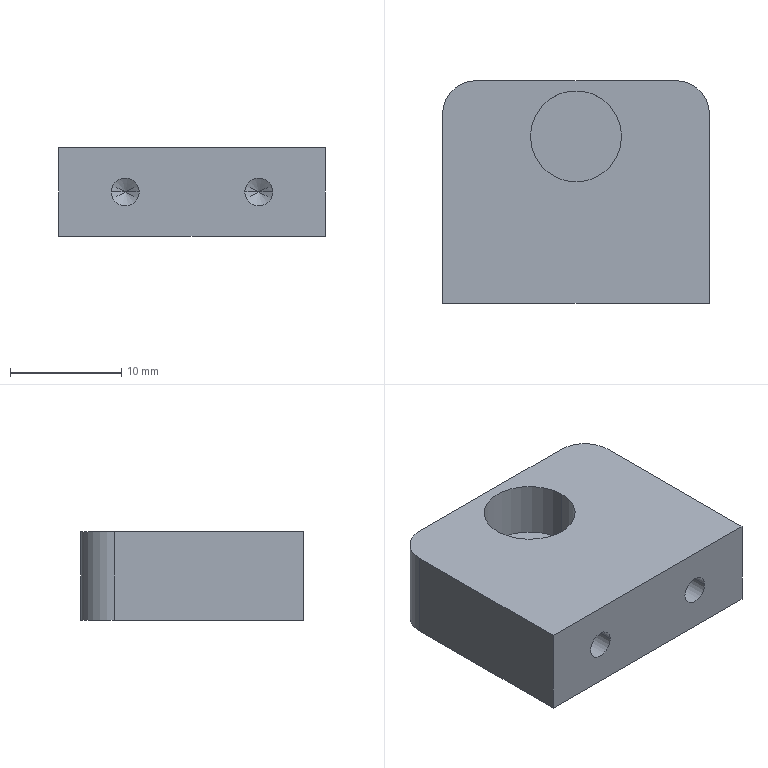Component | SolidWorks | SAWH02-03105A0MountingPlate5-7 | 1 solid | 19 faces | box 24 x 20 x 8 mm | volume 3469 mm3 | cylinder 8 | plane 7 | cone 4 | commonest cylinder face diameters 2.5 x4 8.2 x2 6 x2 | material 6061
build123d program:
from build123d import *

# Parameters (mm, degrees)
SKETCH1_W             = 20
SKETCH1_H             = 24
BOSS_EXTRUDE3_DEPTH   = 8
M3_TAPPED_HOLE1_D     = 2.5
M3_TAPPED_HOLE1_DEPTH = 7.5
M3_TAPPED_HOLE1_TIP   = 0.7511
SKETCH4_R             = 4.1
CUT_EXTRUDE1_DEPTH    = 5
FILLET1_R             = 3


with BuildPart() as part:
    # Sketch1 → Boss-Extrude3 (new body)
    with BuildSketch(Plane(origin=(0, 0, 0), x_dir=(1, 0, 0), z_dir=(0, 1, 0))):
        Rectangle(SKETCH1_W, SKETCH1_H)
    extrude(amount=BOSS_EXTRUDE3_DEPTH)

    # M3 Tapped Hole1
    with Locations(Plane.ZY.offset(10)):
        with Locations((-6, 4), (6, 4)):
            Hole(M3_TAPPED_HOLE1_D / 2, depth=M3_TAPPED_HOLE1_DEPTH)
            with Locations((0, 0, -(M3_TAPPED_HOLE1_DEPTH + M3_TAPPED_HOLE1_TIP / 2))):  # 118° drill point
                Cone(0, M3_TAPPED_HOLE1_D / 2, M3_TAPPED_HOLE1_TIP, mode=Mode.SUBTRACT)

    # Sketch4 → Cut-Extrude1 (cut)
    with BuildSketch(Plane(origin=(0, 8, 0), x_dir=(-1, 0, 0), z_dir=(0, -1, 0))):
        with Locations(Location((-5, 0, 0), (0, 0, 90))):
            Circle(SKETCH4_R)
    extrude(amount=CUT_EXTRUDE1_DEPTH, mode=Mode.SUBTRACT)

    # Fillet1
    fillet1_edges = [part.edges().sort_by_distance(p)[0] for p in [
        (10, 4, 12),
        (10, 4, -12),
    ]]
    fillet(fillet1_edges, radius=FILLET1_R)


solid = part.part

# Placed as in the assembly
solid = solid.moved(Location((81.51, -10.388, -138.792), (90, 90, 0)))
STEP:
#1=COLOUR_RGB('',0.7922,0.8196,0.9333);
#2=FILL_AREA_STYLE_COLOUR('',#1);
#3=FILL_AREA_STYLE('',(#2));
#4=SURFACE_STYLE_FILL_AREA(#3);
#5=SURFACE_SIDE_STYLE('',(#4));
#6=SURFACE_STYLE_USAGE(.BOTH.,#5);
#7=PRESENTATION_STYLE_ASSIGNMENT((#6));
#8=CARTESIAN_POINT('',(3.37,-0.2121,-5.346));
#9=VERTEX_POINT('',#8);
#10=CARTESIAN_POINT('',(3.048,-0.2121,-5.346));
#11=VERTEX_POINT('',#10);
#12=CARTESIAN_POINT('',(3.209,-0.2121,-5.346));
#13=DIRECTION('',(0.,0.,-1.));
#14=DIRECTION('',(-1.,-0.,0.));
#15=AXIS2_PLACEMENT_3D('',#12,#13,#14);
#16=CIRCLE('',#15,0.1614);
#17=EDGE_CURVE('',#9,#11,#16,.T.);
#18=ORIENTED_EDGE('',*,*,#17,.T.);
#19=CARTESIAN_POINT('',(3.048,-0.2121,-5.149));
#20=VERTEX_POINT('',#19);
#21=CARTESIAN_POINT('',(3.048,-0.2121,-5.346));
#22=DIRECTION('',(0.,-0.,1.));
#23=VECTOR('',#22,39.37);
#24=LINE('',#21,#23);
#25=EDGE_CURVE('',#11,#20,#24,.T.);
#26=ORIENTED_EDGE('',*,*,#25,.T.);
#27=CARTESIAN_POINT('',(3.37,-0.2121,-5.149));
#28=VERTEX_POINT('',#27);
#29=CARTESIAN_POINT('',(3.209,-0.2121,-5.149));
#30=DIRECTION('',(0.,0.,-1.));
#31=DIRECTION('',(-1.,-0.,0.));
#32=AXIS2_PLACEMENT_3D('',#29,#30,#31);
#33=CIRCLE('',#32,0.1614);
#34=EDGE_CURVE('',#28,#20,#33,.T.);
#35=ORIENTED_EDGE('',*,*,#34,.F.);
#36=CARTESIAN_POINT('',(3.37,-0.2121,-5.346));
#37=DIRECTION('',(0.,-0.,1.));
#38=VECTOR('',#37,39.37);
#39=LINE('',#36,#38);
#40=EDGE_CURVE('',#9,#28,#39,.T.);
#41=ORIENTED_EDGE('',*,*,#40,.F.);
#42=EDGE_LOOP('',(#18,#26,#35,#41));
#43=FACE_OUTER_BOUND('',#42,.T.);
#44=CARTESIAN_POINT('',(3.209,-0.2121,-5.346));
#45=DIRECTION('',(0.,-0.,1.));
#46=DIRECTION('',(1.,0.,0.));
#47=AXIS2_PLACEMENT_3D('',#44,#45,#46);
#48=CYLINDRICAL_SURFACE('',#47,0.1614);
#49=ADVANCED_FACE('',(#43),#48,.F.);
#50=CARTESIAN_POINT('',(2.924,-0.5074,-5.307));
#51=VERTEX_POINT('',#50);
#52=CARTESIAN_POINT('',(3.022,-0.5074,-5.307));
#53=VERTEX_POINT('',#52);
#54=CARTESIAN_POINT('',(2.973,-0.5074,-5.307));
#55=DIRECTION('',(0.,-1.,0.));
#56=DIRECTION('',(1.,0.,0.));
#57=AXIS2_PLACEMENT_3D('',#54,#55,#56);
#58=CIRCLE('',#57,0.04921);
#59=EDGE_CURVE('',#51,#53,#58,.T.);
#60=ORIENTED_EDGE('',*,*,#59,.F.);
#61=CARTESIAN_POINT('',(2.924,-0.8027,-5.307));
#62=VERTEX_POINT('',#61);
#63=CARTESIAN_POINT('',(2.924,-0.8027,-5.307));
#64=DIRECTION('',(0.,-1.,0.));
#65=VECTOR('',#64,39.37);
#66=LINE('',#63,#65);
#67=EDGE_CURVE('',#51,#62,#66,.T.);
#68=ORIENTED_EDGE('',*,*,#67,.T.);
#69=CARTESIAN_POINT('',(3.022,-0.8027,-5.307));
#70=VERTEX_POINT('',#69);
#71=CARTESIAN_POINT('',(2.973,-0.8027,-5.307));
#72=DIRECTION('',(0.,-1.,0.));
#73=DIRECTION('',(1.,0.,0.));
#74=AXIS2_PLACEMENT_3D('',#71,#72,#73);
#75=CIRCLE('',#74,0.04921);
#76=EDGE_CURVE('',#62,#70,#75,.T.);
#77=ORIENTED_EDGE('',*,*,#76,.T.);
#78=CARTESIAN_POINT('',(3.022,-0.8027,-5.307));
#79=DIRECTION('',(0.,-1.,0.));
#80=VECTOR('',#79,39.37);
#81=LINE('',#78,#80);
#82=EDGE_CURVE('',#53,#70,#81,.T.);
#83=ORIENTED_EDGE('',*,*,#82,.F.);
#84=EDGE_LOOP('',(#60,#68,#77,#83));
#85=FACE_OUTER_BOUND('',#84,.T.);
#86=CARTESIAN_POINT('',(2.973,-0.8027,-5.307));
#87=DIRECTION('',(0.,-1.,0.));
#88=DIRECTION('',(1.,0.,0.));
#89=AXIS2_PLACEMENT_3D('',#86,#87,#88);
#90=CYLINDRICAL_SURFACE('',#89,0.04921);
#91=ADVANCED_FACE('',(#85),#90,.F.);
#92=CARTESIAN_POINT('',(2.973,-0.4778,-5.307));
#93=VERTEX_POINT('',#92);
#94=CARTESIAN_POINT('',(3.022,-0.5074,-5.307));
#95=DIRECTION('',(0.8572,-0.515,0.));
#96=VECTOR('',#95,39.37);
#97=LINE('',#94,#96);
#98=EDGE_CURVE('',#93,#53,#97,.T.);
#99=ORIENTED_EDGE('',*,*,#98,.F.);
#100=CARTESIAN_POINT('',(2.924,-0.5074,-5.307));
#101=DIRECTION('',(-0.8572,-0.515,0.));
#102=VECTOR('',#101,39.37);
#103=LINE('',#100,#102);
#104=EDGE_CURVE('',#93,#51,#103,.T.);
#105=ORIENTED_EDGE('',*,*,#104,.T.);
#106=ORIENTED_EDGE('',*,*,#59,.T.);
#107=EDGE_LOOP('',(#99,#105,#106));
#108=FACE_OUTER_BOUND('',#107,.T.);
#109=CARTESIAN_POINT('',(2.973,-0.5074,-5.307));
#110=DIRECTION('',(0.,-1.,0.));
#111=DIRECTION('',(1.,0.,0.));
#112=AXIS2_PLACEMENT_3D('',#109,#110,#111);
#113=CONICAL_SURFACE('',#112,0.04921,1.03);
#114=ADVANCED_FACE('',(#108),#113,.F.);
#115=CARTESIAN_POINT('',(3.396,-0.5074,-5.307));
#116=VERTEX_POINT('',#115);
#117=CARTESIAN_POINT('',(3.494,-0.5074,-5.307));
#118=VERTEX_POINT('',#117);
#119=CARTESIAN_POINT('',(3.445,-0.5074,-5.307));
#120=DIRECTION('',(0.,-1.,0.));
#121=DIRECTION('',(1.,0.,0.));
#122=AXIS2_PLACEMENT_3D('',#119,#120,#121);
#123=CIRCLE('',#122,0.04921);
#124=EDGE_CURVE('',#116,#118,#123,.T.);
#125=ORIENTED_EDGE('',*,*,#124,.F.);
#126=CARTESIAN_POINT('',(3.396,-0.8027,-5.307));
#127=VERTEX_POINT('',#126);
#128=CARTESIAN_POINT('',(3.396,-0.8027,-5.307));
#129=DIRECTION('',(0.,-1.,0.));
#130=VECTOR('',#129,39.37);
#131=LINE('',#128,#130);
#132=EDGE_CURVE('',#116,#127,#131,.T.);
#133=ORIENTED_EDGE('',*,*,#132,.T.);
#134=CARTESIAN_POINT('',(3.494,-0.8027,-5.307));
#135=VERTEX_POINT('',#134);
#136=CARTESIAN_POINT('',(3.445,-0.8027,-5.307));
#137=DIRECTION('',(0.,-1.,0.));
#138=DIRECTION('',(1.,0.,0.));
#139=AXIS2_PLACEMENT_3D('',#136,#137,#138);
#140=CIRCLE('',#139,0.04921);
#141=EDGE_CURVE('',#127,#135,#140,.T.);
#142=ORIENTED_EDGE('',*,*,#141,.T.);
#143=CARTESIAN_POINT('',(3.494,-0.8027,-5.307));
#144=DIRECTION('',(0.,-1.,0.));
#145=VECTOR('',#144,39.37);
#146=LINE('',#143,#145);
#147=EDGE_CURVE('',#118,#135,#146,.T.);
#148=ORIENTED_EDGE('',*,*,#147,.F.);
#149=EDGE_LOOP('',(#125,#133,#142,#148));
#150=FACE_OUTER_BOUND('',#149,.T.);
#151=CARTESIAN_POINT('',(3.445,-0.8027,-5.307));
#152=DIRECTION('',(0.,-1.,0.));
#153=DIRECTION('',(1.,0.,0.));
#154=AXIS2_PLACEMENT_3D('',#151,#152,#153);
#155=CYLINDRICAL_SURFACE('',#154,0.04921);
#156=ADVANCED_FACE('',(#150),#155,.F.);
#157=CARTESIAN_POINT('',(3.445,-0.4778,-5.307));
#158=VERTEX_POINT('',#157);
#159=CARTESIAN_POINT('',(3.494,-0.5074,-5.307));
#160=DIRECTION('',(0.8572,-0.515,0.));
#161=VECTOR('',#160,39.37);
#162=LINE('',#159,#161);
#163=EDGE_CURVE('',#158,#118,#162,.T.);
#164=ORIENTED_EDGE('',*,*,#163,.F.);
#165=CARTESIAN_POINT('',(3.396,-0.5074,-5.307));
#166=DIRECTION('',(-0.8572,-0.515,0.));
#167=VECTOR('',#166,39.37);
#168=LINE('',#165,#167);
#169=EDGE_CURVE('',#158,#116,#168,.T.);
#170=ORIENTED_EDGE('',*,*,#169,.T.);
#171=ORIENTED_EDGE('',*,*,#124,.T.);
#172=EDGE_LOOP('',(#164,#170,#171));
#173=FACE_OUTER_BOUND('',#172,.T.);
#174=CARTESIAN_POINT('',(3.445,-0.5074,-5.307));
#175=DIRECTION('',(0.,-1.,0.));
#176=DIRECTION('',(1.,0.,0.));
#177=AXIS2_PLACEMENT_3D('',#174,#175,#176);
#178=CONICAL_SURFACE('',#177,0.04921,1.03);
#179=ADVANCED_FACE('',(#173),#178,.F.);
#180=CARTESIAN_POINT('',(3.563,-0.01526,-5.149));
#181=VERTEX_POINT('',#180);
#182=CARTESIAN_POINT('',(2.855,-0.01526,-5.149));
#183=VERTEX_POINT('',#182);
#184=CARTESIAN_POINT('',(3.682,-0.01526,-5.149));
#185=DIRECTION('',(-1.,-0.,0.));
#186=VECTOR('',#185,39.37);
#187=LINE('',#184,#186);
#188=EDGE_CURVE('',#181,#183,#187,.T.);
#189=ORIENTED_EDGE('',*,*,#188,.F.);
#190=CARTESIAN_POINT('',(3.563,-0.01526,-5.464));
#191=VERTEX_POINT('',#190);
#192=CARTESIAN_POINT('',(3.563,-0.01526,-5.149));
#193=DIRECTION('',(0.,0.,-1.));
#194=VECTOR('',#193,39.37);
#195=LINE('',#192,#194);
#196=EDGE_CURVE('',#181,#191,#195,.T.);
#197=ORIENTED_EDGE('',*,*,#196,.T.);
#198=CARTESIAN_POINT('',(2.855,-0.01526,-5.464));
#199=VERTEX_POINT('',#198);
#200=CARTESIAN_POINT('',(3.682,-0.01526,-5.464));
#201=DIRECTION('',(-1.,-0.,0.));
#202=VECTOR('',#201,39.37);
#203=LINE('',#200,#202);
#204=EDGE_CURVE('',#191,#199,#203,.T.);
#205=ORIENTED_EDGE('',*,*,#204,.T.);
#206=CARTESIAN_POINT('',(2.855,-0.01526,-5.149));
#207=DIRECTION('',(0.,-0.,1.));
#208=VECTOR('',#207,39.37);
#209=LINE('',#206,#208);
#210=EDGE_CURVE('',#199,#183,#209,.T.);
#211=ORIENTED_EDGE('',*,*,#210,.T.);
#212=EDGE_LOOP('',(#189,#197,#205,#211));
#213=FACE_OUTER_BOUND('',#212,.T.);
#214=CARTESIAN_POINT('',(3.682,-0.01526,-5.149));
#215=DIRECTION('',(0.,-1.,0.));
#216=DIRECTION('',(1.,0.,0.));
#217=AXIS2_PLACEMENT_3D('',#214,#215,#216);
#218=PLANE('',#217);
#219=ADVANCED_FACE('',(#213),#218,.F.);
#220=CARTESIAN_POINT('',(2.737,-0.1334,-5.149));
#221=VERTEX_POINT('',#220);
#222=CARTESIAN_POINT('',(2.737,-0.8027,-5.149));
#223=VERTEX_POINT('',#222);
#224=CARTESIAN_POINT('',(2.737,-0.8027,-5.149));
#225=DIRECTION('',(0.,-1.,0.));
#226=VECTOR('',#225,39.37);
#227=LINE('',#224,#226);
#228=EDGE_CURVE('',#221,#223,#227,.T.);
#229=ORIENTED_EDGE('',*,*,#228,.F.);
#230=CARTESIAN_POINT('',(2.737,-0.1334,-5.464));
#231=VERTEX_POINT('',#230);
#232=CARTESIAN_POINT('',(2.737,-0.1334,-5.149));
#233=DIRECTION('',(0.,0.,-1.));
#234=VECTOR('',#233,39.37);
#235=LINE('',#232,#234);
#236=EDGE_CURVE('',#221,#231,#235,.T.);
#237=ORIENTED_EDGE('',*,*,#236,.T.);
#238=CARTESIAN_POINT('',(2.737,-0.8027,-5.464));
#239=VERTEX_POINT('',#238);
#240=CARTESIAN_POINT('',(2.737,-0.8027,-5.464));
#241=DIRECTION('',(0.,-1.,0.));
#242=VECTOR('',#241,39.37);
#243=LINE('',#240,#242);
#244=EDGE_CURVE('',#231,#239,#243,.T.);
#245=ORIENTED_EDGE('',*,*,#244,.T.);
#246=CARTESIAN_POINT('',(2.737,-0.8027,-5.149));
#247=DIRECTION('',(0.,0.,-1.));
#248=VECTOR('',#247,39.37);
#249=LINE('',#246,#248);
#250=EDGE_CURVE('',#223,#239,#249,.T.);
#251=ORIENTED_EDGE('',*,*,#250,.F.);
#252=EDGE_LOOP('',(#229,#237,#245,#251));
#253=FACE_OUTER_BOUND('',#252,.T.);
#254=CARTESIAN_POINT('',(2.737,-0.8027,-5.149));
#255=DIRECTION('',(1.,0.,0.));
#256=DIRECTION('',(-0.,1.,-0.));
#257=AXIS2_PLACEMENT_3D('',#254,#255,#256);
#258=PLANE('',#257);
#259=ADVANCED_FACE('',(#253),#258,.F.);
#260=CARTESIAN_POINT('',(2.973,-0.8027,-5.307));
#261=DIRECTION('',(0.,-1.,0.));
#262=DIRECTION('',(1.,0.,0.));
#263=AXIS2_PLACEMENT_3D('',#260,#261,#262);
#264=CIRCLE('',#263,0.04921);
#265=EDGE_CURVE('',#70,#62,#264,.T.);
#266=ORIENTED_EDGE('',*,*,#265,.F.);
#267=ORIENTED_EDGE('',*,*,#76,.F.);
#268=EDGE_LOOP('',(#266,#267));
#269=FACE_BOUND('',#268,.T.);
#270=CARTESIAN_POINT('',(3.445,-0.8027,-5.307));
#271=DIRECTION('',(0.,-1.,0.));
#272=DIRECTION('',(1.,0.,0.));
#273=AXIS2_PLACEMENT_3D('',#270,#271,#272);
#274=CIRCLE('',#273,0.04921);
#275=EDGE_CURVE('',#135,#127,#274,.T.);
#276=ORIENTED_EDGE('',*,*,#275,.F.);
#277=ORIENTED_EDGE('',*,*,#141,.F.);
#278=EDGE_LOOP('',(#276,#277));
#279=FACE_BOUND('',#278,.T.);
#280=CARTESIAN_POINT('',(3.682,-0.8027,-5.464));
#281=VERTEX_POINT('',#280);
#282=CARTESIAN_POINT('',(3.682,-0.8027,-5.464));
#283=DIRECTION('',(1.,0.,0.));
#284=VECTOR('',#283,39.37);
#285=LINE('',#282,#284);
#286=EDGE_CURVE('',#239,#281,#285,.T.);
#287=ORIENTED_EDGE('',*,*,#286,.T.);
#288=CARTESIAN_POINT('',(3.682,-0.8027,-5.149));
#289=VERTEX_POINT('',#288);
#290=CARTESIAN_POINT('',(3.682,-0.8027,-5.149));
#291=DIRECTION('',(0.,0.,-1.));
#292=VECTOR('',#291,39.37);
#293=LINE('',#290,#292);
#294=EDGE_CURVE('',#289,#281,#293,.T.);
#295=ORIENTED_EDGE('',*,*,#294,.F.);
#296=CARTESIAN_POINT('',(3.682,-0.8027,-5.149));
#297=DIRECTION('',(1.,0.,0.));
#298=VECTOR('',#297,39.37);
#299=LINE('',#296,#298);
#300=EDGE_CURVE('',#223,#289,#299,.T.);
#301=ORIENTED_EDGE('',*,*,#300,.F.);
#302=ORIENTED_EDGE('',*,*,#250,.T.);
#303=EDGE_LOOP('',(#287,#295,#301,#302));
#304=FACE_OUTER_BOUND('',#303,.T.);
#305=CARTESIAN_POINT('',(3.682,-0.8027,-5.149));
#306=DIRECTION('',(-0.,1.,-0.));
#307=DIRECTION('',(-1.,-0.,0.));
#308=AXIS2_PLACEMENT_3D('',#305,#306,#307);
#309=PLANE('',#308);
#310=ADVANCED_FACE('',(#269,#279,#304),#309,.F.);
#311=CARTESIAN_POINT('',(3.682,-0.1334,-5.464));
#312=VERTEX_POINT('',#311);
#313=CARTESIAN_POINT('',(3.682,-0.8027,-5.464));
#314=DIRECTION('',(-0.,1.,-0.));
#315=VECTOR('',#314,39.37);
#316=LINE('',#313,#315);
#317=EDGE_CURVE('',#281,#312,#316,.T.);
#318=ORIENTED_EDGE('',*,*,#317,.T.);
#319=CARTESIAN_POINT('',(3.682,-0.1334,-5.149));
#320=VERTEX_POINT('',#319);
#321=CARTESIAN_POINT('',(3.682,-0.1334,-5.149));
#322=DIRECTION('',(0.,-0.,1.));
#323=VECTOR('',#322,39.37);
#324=LINE('',#321,#323);
#325=EDGE_CURVE('',#312,#320,#324,.T.);
#326=ORIENTED_EDGE('',*,*,#325,.T.);
#327=CARTESIAN_POINT('',(3.682,-0.8027,-5.149));
#328=DIRECTION('',(-0.,1.,-0.));
#329=VECTOR('',#328,39.37);
#330=LINE('',#327,#329);
#331=EDGE_CURVE('',#289,#320,#330,.T.);
#332=ORIENTED_EDGE('',*,*,#331,.F.);
#333=ORIENTED_EDGE('',*,*,#294,.T.);
#334=EDGE_LOOP('',(#318,#326,#332,#333));
#335=FACE_OUTER_BOUND('',#334,.T.);
#336=CARTESIAN_POINT('',(3.682,-0.8027,-5.149));
#337=DIRECTION('',(-1.,-0.,-0.));
#338=DIRECTION('',(0.,-1.,0.));
#339=AXIS2_PLACEMENT_3D('',#336,#337,#338);
#340=PLANE('',#339);
#341=ADVANCED_FACE('',(#335),#340,.F.);
#342=ORIENTED_EDGE('',*,*,#34,.T.);
#343=CARTESIAN_POINT('',(3.209,-0.2121,-5.149));
#344=DIRECTION('',(0.,0.,-1.));
#345=DIRECTION('',(-1.,-0.,0.));
#346=AXIS2_PLACEMENT_3D('',#343,#344,#345);
#347=CIRCLE('',#346,0.1614);
#348=EDGE_CURVE('',#20,#28,#347,.T.);
#349=ORIENTED_EDGE('',*,*,#348,.T.);
#350=EDGE_LOOP('',(#342,#349));
#351=FACE_BOUND('',#350,.T.);
#352=ORIENTED_EDGE('',*,*,#331,.T.);
#353=CARTESIAN_POINT('',(3.563,-0.1334,-5.149));
#354=DIRECTION('',(0.,-0.,1.));
#355=DIRECTION('',(-1.,-0.,0.));
#356=AXIS2_PLACEMENT_3D('',#353,#354,#355);
#357=CIRCLE('',#356,0.1181);
#358=EDGE_CURVE('',#320,#181,#357,.T.);
#359=ORIENTED_EDGE('',*,*,#358,.T.);
#360=ORIENTED_EDGE('',*,*,#188,.T.);
#361=CARTESIAN_POINT('',(2.855,-0.1334,-5.149));
#362=DIRECTION('',(0.,-0.,1.));
#363=DIRECTION('',(-1.,0.,0.));
#364=AXIS2_PLACEMENT_3D('',#361,#362,#363);
#365=CIRCLE('',#364,0.1181);
#366=EDGE_CURVE('',#183,#221,#365,.T.);
#367=ORIENTED_EDGE('',*,*,#366,.T.);
#368=ORIENTED_EDGE('',*,*,#228,.T.);
#369=ORIENTED_EDGE('',*,*,#300,.T.);
#370=EDGE_LOOP('',(#352,#359,#360,#367,#368,#369));
#371=FACE_OUTER_BOUND('',#370,.T.);
#372=CARTESIAN_POINT('',(3.209,-0.409,-5.149));
#373=DIRECTION('',(-0.,0.,-1.));
#374=DIRECTION('',(-1.,-0.,0.));
#375=AXIS2_PLACEMENT_3D('',#372,#373,#374);
#376=PLANE('',#375);
#377=ADVANCED_FACE('',(#351,#371),#376,.F.);
#378=ORIENTED_EDGE('',*,*,#204,.F.);
#379=CARTESIAN_POINT('',(3.563,-0.1334,-5.464));
#380=DIRECTION('',(0.,0.,-1.));
#381=DIRECTION('',(-1.,-0.,0.));
#382=AXIS2_PLACEMENT_3D('',#379,#380,#381);
#383=CIRCLE('',#382,0.1181);
#384=EDGE_CURVE('',#191,#312,#383,.T.);
#385=ORIENTED_EDGE('',*,*,#384,.T.);
#386=ORIENTED_EDGE('',*,*,#317,.F.);
#387=ORIENTED_EDGE('',*,*,#286,.F.);
#388=ORIENTED_EDGE('',*,*,#244,.F.);
#389=CARTESIAN_POINT('',(2.855,-0.1334,-5.464));
#390=DIRECTION('',(0.,0.,-1.));
#391=DIRECTION('',(-1.,-0.,0.));
#392=AXIS2_PLACEMENT_3D('',#389,#390,#391);
#393=CIRCLE('',#392,0.1181);
#394=EDGE_CURVE('',#231,#199,#393,.T.);
#395=ORIENTED_EDGE('',*,*,#394,.T.);
#396=EDGE_LOOP('',(#378,#385,#386,#387,#388,#395));
#397=FACE_OUTER_BOUND('',#396,.T.);
#398=CARTESIAN_POINT('',(3.209,-0.409,-5.464));
#399=DIRECTION('',(-0.,0.,-1.));
#400=DIRECTION('',(-1.,-0.,0.));
#401=AXIS2_PLACEMENT_3D('',#398,#399,#400);
#402=PLANE('',#401);
#403=ADVANCED_FACE('',(#397),#402,.T.);
#404=ORIENTED_EDGE('',*,*,#169,.F.);
#405=ORIENTED_EDGE('',*,*,#163,.T.);
#406=CARTESIAN_POINT('',(3.445,-0.5074,-5.307));
#407=DIRECTION('',(0.,-1.,0.));
#408=DIRECTION('',(1.,0.,0.));
#409=AXIS2_PLACEMENT_3D('',#406,#407,#408);
#410=CIRCLE('',#409,0.04921);
#411=EDGE_CURVE('',#118,#116,#410,.T.);
#412=ORIENTED_EDGE('',*,*,#411,.T.);
#413=EDGE_LOOP('',(#404,#405,#412));
#414=FACE_OUTER_BOUND('',#413,.T.);
#415=CARTESIAN_POINT('',(3.445,-0.5074,-5.307));
#416=DIRECTION('',(0.,-1.,0.));
#417=DIRECTION('',(1.,0.,0.));
#418=AXIS2_PLACEMENT_3D('',#415,#416,#417);
#419=CONICAL_SURFACE('',#418,0.04921,1.03);
#420=ADVANCED_FACE('',(#414),#419,.F.);
#421=ORIENTED_EDGE('',*,*,#132,.F.);
#422=ORIENTED_EDGE('',*,*,#411,.F.);
#423=ORIENTED_EDGE('',*,*,#147,.T.);
#424=ORIENTED_EDGE('',*,*,#275,.T.);
#425=EDGE_LOOP('',(#421,#422,#423,#424));
#426=FACE_OUTER_BOUND('',#425,.T.);
#427=CARTESIAN_POINT('',(3.445,-0.8027,-5.307));
#428=DIRECTION('',(0.,-1.,0.));
#429=DIRECTION('',(1.,0.,0.));
#430=AXIS2_PLACEMENT_3D('',#427,#428,#429);
#431=CYLINDRICAL_SURFACE('',#430,0.04921);
#432=ADVANCED_FACE('',(#426),#431,.F.);
#433=ORIENTED_EDGE('',*,*,#104,.F.);
#434=ORIENTED_EDGE('',*,*,#98,.T.);
#435=CARTESIAN_POINT('',(2.973,-0.5074,-5.307));
#436=DIRECTION('',(0.,-1.,0.));
#437=DIRECTION('',(1.,0.,0.));
#438=AXIS2_PLACEMENT_3D('',#435,#436,#437);
#439=CIRCLE('',#438,0.04921);
#440=EDGE_CURVE('',#53,#51,#439,.T.);
#441=ORIENTED_EDGE('',*,*,#440,.T.);
#442=EDGE_LOOP('',(#433,#434,#441));
#443=FACE_OUTER_BOUND('',#442,.T.);
#444=CARTESIAN_POINT('',(2.973,-0.5074,-5.307));
#445=DIRECTION('',(0.,-1.,0.));
#446=DIRECTION('',(1.,0.,0.));
#447=AXIS2_PLACEMENT_3D('',#444,#445,#446);
#448=CONICAL_SURFACE('',#447,0.04921,1.03);
#449=ADVANCED_FACE('',(#443),#448,.F.);
#450=ORIENTED_EDGE('',*,*,#67,.F.);
#451=ORIENTED_EDGE('',*,*,#440,.F.);
#452=ORIENTED_EDGE('',*,*,#82,.T.);
#453=ORIENTED_EDGE('',*,*,#265,.T.);
#454=EDGE_LOOP('',(#450,#451,#452,#453));
#455=FACE_OUTER_BOUND('',#454,.T.);
#456=CARTESIAN_POINT('',(2.973,-0.8027,-5.307));
#457=DIRECTION('',(0.,-1.,0.));
#458=DIRECTION('',(1.,0.,0.));
#459=AXIS2_PLACEMENT_3D('',#456,#457,#458);
#460=CYLINDRICAL_SURFACE('',#459,0.04921);
#461=ADVANCED_FACE('',(#455),#460,.F.);
#462=ORIENTED_EDGE('',*,*,#25,.F.);
#463=CARTESIAN_POINT('',(3.209,-0.2121,-5.346));
#464=DIRECTION('',(0.,0.,-1.));
#465=DIRECTION('',(-1.,-0.,0.));
#466=AXIS2_PLACEMENT_3D('',#463,#464,#465);
#467=CIRCLE('',#466,0.1614);
#468=EDGE_CURVE('',#11,#9,#467,.T.);
#469=ORIENTED_EDGE('',*,*,#468,.T.);
#470=ORIENTED_EDGE('',*,*,#40,.T.);
#471=ORIENTED_EDGE('',*,*,#348,.F.);
#472=EDGE_LOOP('',(#462,#469,#470,#471));
#473=FACE_OUTER_BOUND('',#472,.T.);
#474=CARTESIAN_POINT('',(3.209,-0.2121,-5.346));
#475=DIRECTION('',(0.,-0.,1.));
#476=DIRECTION('',(1.,0.,0.));
#477=AXIS2_PLACEMENT_3D('',#474,#475,#476);
#478=CYLINDRICAL_SURFACE('',#477,0.1614);
#479=ADVANCED_FACE('',(#473),#478,.F.);
#480=ORIENTED_EDGE('',*,*,#17,.F.);
#481=ORIENTED_EDGE('',*,*,#468,.F.);
#482=EDGE_LOOP('',(#480,#481));
#483=FACE_OUTER_BOUND('',#482,.T.);
#484=CARTESIAN_POINT('',(3.209,-0.2121,-5.346));
#485=DIRECTION('',(-0.,0.,-1.));
#486=DIRECTION('',(-1.,-0.,0.));
#487=AXIS2_PLACEMENT_3D('',#484,#485,#486);
#488=PLANE('',#487);
#489=ADVANCED_FACE('',(#483),#488,.F.);
#490=ORIENTED_EDGE('',*,*,#358,.F.);
#491=ORIENTED_EDGE('',*,*,#325,.F.);
#492=ORIENTED_EDGE('',*,*,#384,.F.);
#493=ORIENTED_EDGE('',*,*,#196,.F.);
#494=EDGE_LOOP('',(#490,#491,#492,#493));
#495=FACE_OUTER_BOUND('',#494,.T.);
#496=CARTESIAN_POINT('',(3.563,-0.1334,-5.149));
#497=DIRECTION('',(0.,0.,-1.));
#498=DIRECTION('',(-1.,-0.,0.));
#499=AXIS2_PLACEMENT_3D('',#496,#497,#498);
#500=CYLINDRICAL_SURFACE('',#499,0.1181);
#501=ADVANCED_FACE('',(#495),#500,.T.);
#502=ORIENTED_EDGE('',*,*,#366,.F.);
#503=ORIENTED_EDGE('',*,*,#210,.F.);
#504=ORIENTED_EDGE('',*,*,#394,.F.);
#505=ORIENTED_EDGE('',*,*,#236,.F.);
#506=EDGE_LOOP('',(#502,#503,#504,#505));
#507=FACE_OUTER_BOUND('',#506,.T.);
#508=CARTESIAN_POINT('',(2.855,-0.1334,-5.149));
#509=DIRECTION('',(0.,0.,-1.));
#510=DIRECTION('',(-1.,-0.,0.));
#511=AXIS2_PLACEMENT_3D('',#508,#509,#510);
#512=CYLINDRICAL_SURFACE('',#511,0.1181);
#513=ADVANCED_FACE('',(#507),#512,.T.);
#514=CLOSED_SHELL('',(#49,#91,#114,#156,#179,#219,#259,#310,#341,#377,#403,#420,#432,#449,#461,#479,#489,#501,#513));
#515=MANIFOLD_SOLID_BREP('',#514);
#516=STYLED_ITEM('',(#7),#515);
#517=(LENGTH_UNIT()NAMED_UNIT(*)SI_UNIT($,.METRE.));
#518=LENGTH_MEASURE_WITH_UNIT(LENGTH_MEASURE(0.0254),#517);
#519=DIMENSIONAL_EXPONENTS(1.,0.,0.,0.,0.,0.,0.);
#520=(CONVERSION_BASED_UNIT('',#518)LENGTH_UNIT()NAMED_UNIT(#519));
#521=UNCERTAINTY_MEASURE_WITH_UNIT(LENGTH_MEASURE(0.00001),#520,'','');
#522=(NAMED_UNIT(*)PLANE_ANGLE_UNIT()SI_UNIT($,.RADIAN.));
#523=(NAMED_UNIT(*)SI_UNIT($,.STERADIAN.)SOLID_ANGLE_UNIT());
#524=(GEOMETRIC_REPRESENTATION_CONTEXT(3)GLOBAL_UNCERTAINTY_ASSIGNED_CONTEXT((#521))GLOBAL_UNIT_ASSIGNED_CONTEXT((#520,#522,#523))REPRESENTATION_CONTEXT('',''));
#525=MECHANICAL_DESIGN_GEOMETRIC_PRESENTATION_REPRESENTATION('',(#516),#524);
#526=CARTESIAN_POINT('',(0.,0.,0.));
#527=DIRECTION('',(0.,0.,1.));
#528=DIRECTION('',(1.,0.,0.));
#529=AXIS2_PLACEMENT_3D('',#526,#527,#528);
#530=(LENGTH_UNIT()NAMED_UNIT(*)SI_UNIT($,.METRE.));
#531=LENGTH_MEASURE_WITH_UNIT(LENGTH_MEASURE(0.0254),#530);
#532=DIMENSIONAL_EXPONENTS(1.,0.,0.,0.,0.,0.,0.);
#533=(CONVERSION_BASED_UNIT('',#531)LENGTH_UNIT()NAMED_UNIT(#532));
#534=UNCERTAINTY_MEASURE_WITH_UNIT(LENGTH_MEASURE(0.00001),#533,'','');
#535=(NAMED_UNIT(*)PLANE_ANGLE_UNIT()SI_UNIT($,.RADIAN.));
#536=(NAMED_UNIT(*)SI_UNIT($,.STERADIAN.)SOLID_ANGLE_UNIT());
#537=(GEOMETRIC_REPRESENTATION_CONTEXT(3)GLOBAL_UNCERTAINTY_ASSIGNED_CONTEXT((#534))GLOBAL_UNIT_ASSIGNED_CONTEXT((#533,#535,#536))REPRESENTATION_CONTEXT('',''));
#538=ADVANCED_BREP_SHAPE_REPRESENTATION('',(#515,#529),#537);
#539=PRESENTATION_LAYER_ASSIGNMENT('','',(#516));